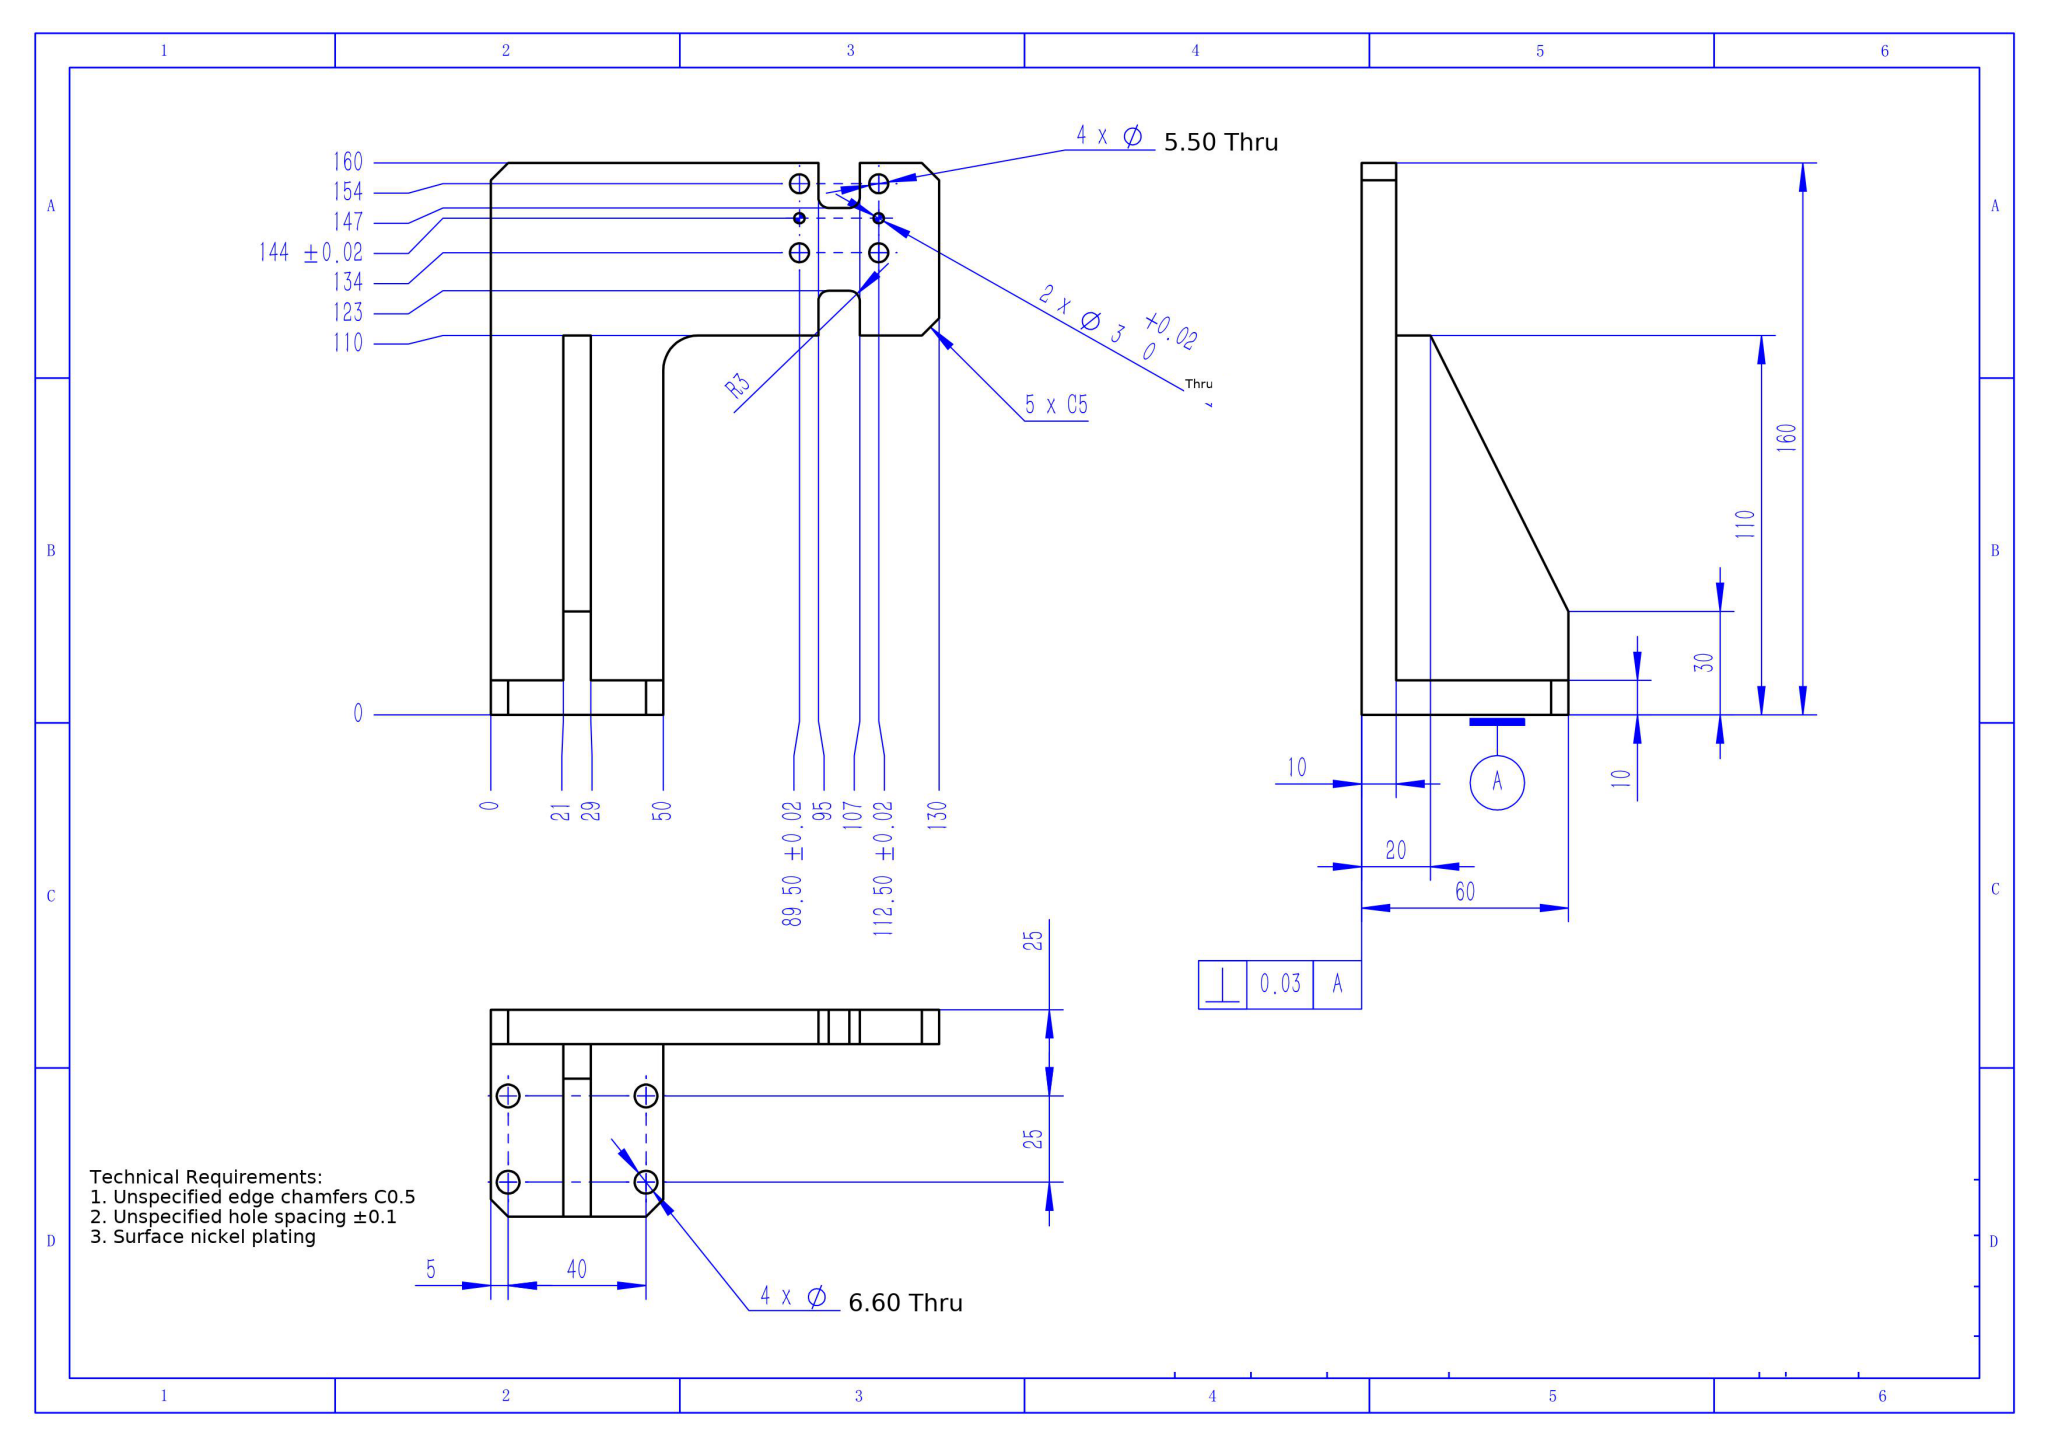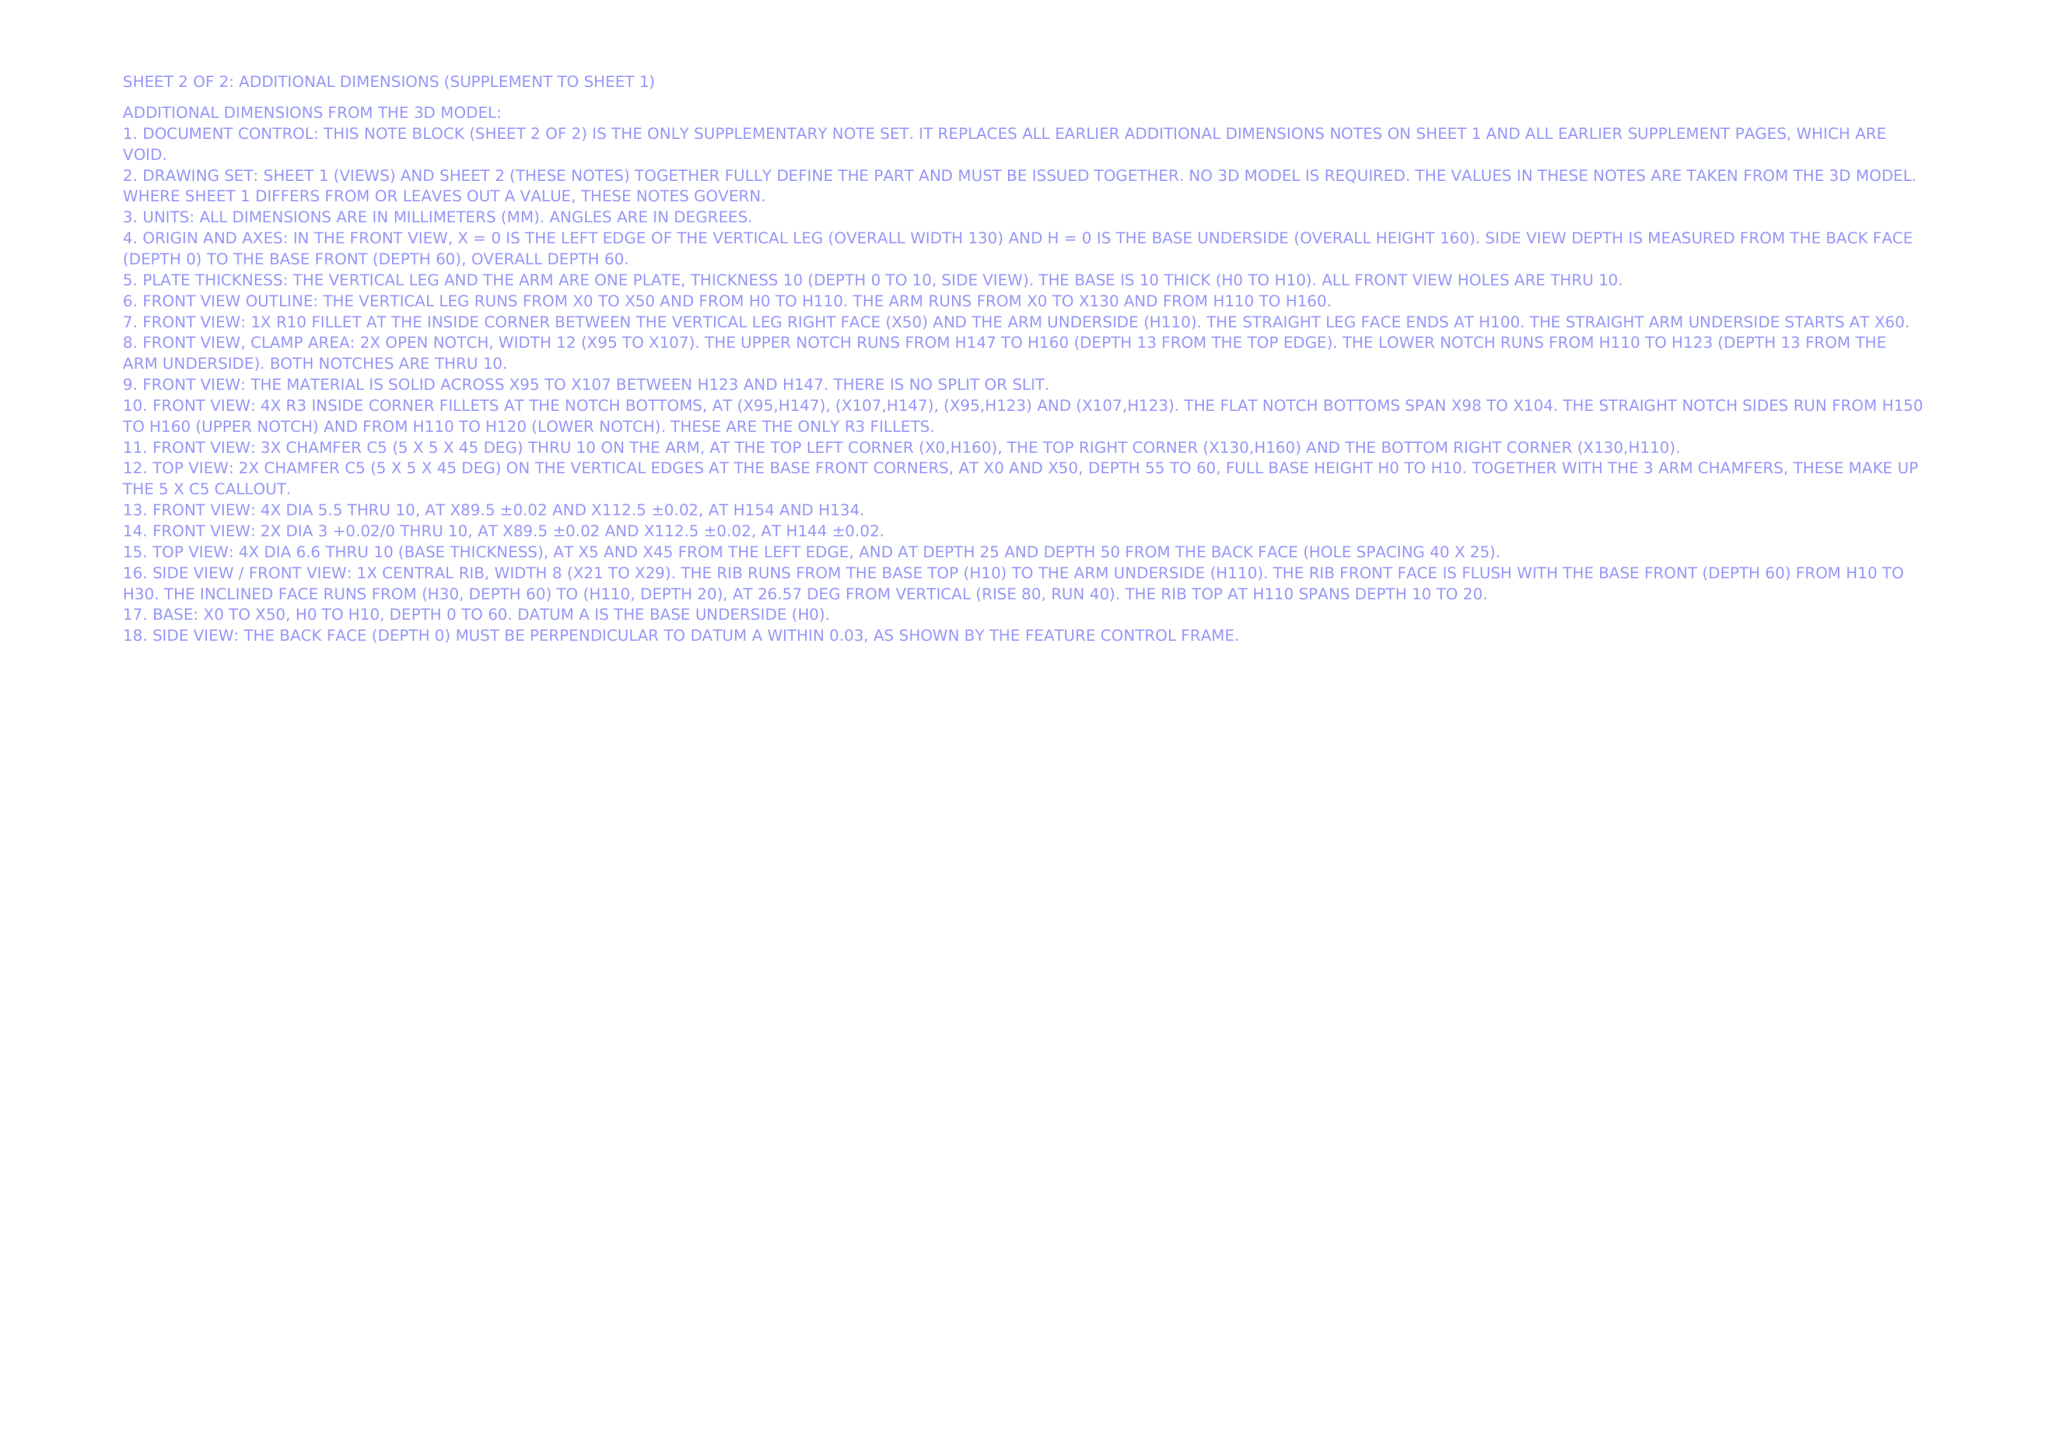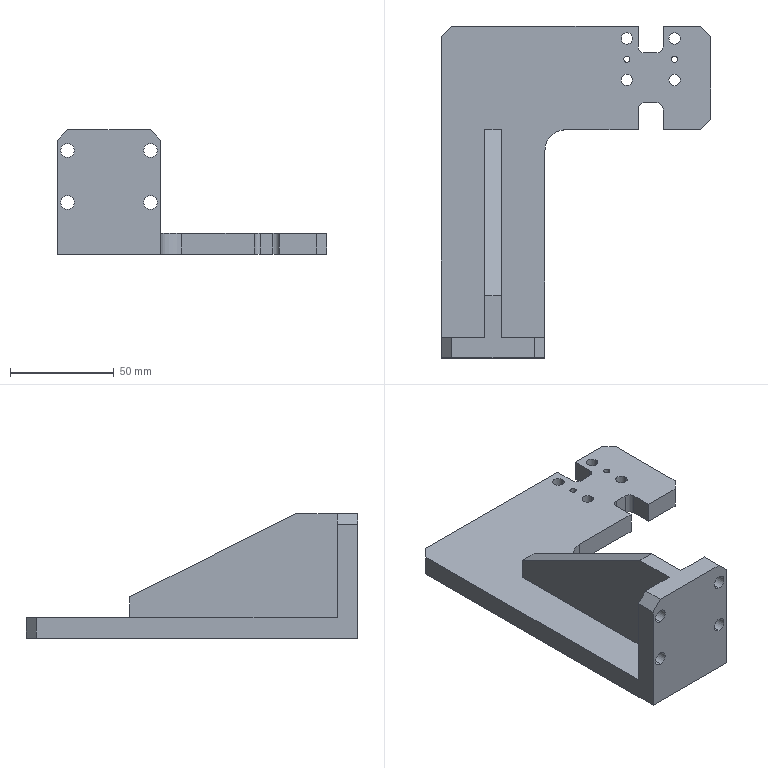Part | NX | mm | 1 solid | 53 faces | box 130 x 160 x 60 mm | volume 166287 mm3 | plane 28 | cylinder 25 | commonest cylinder face diameters 6.6 x8 5.5 x8 3 x4 6 x4 20 x1